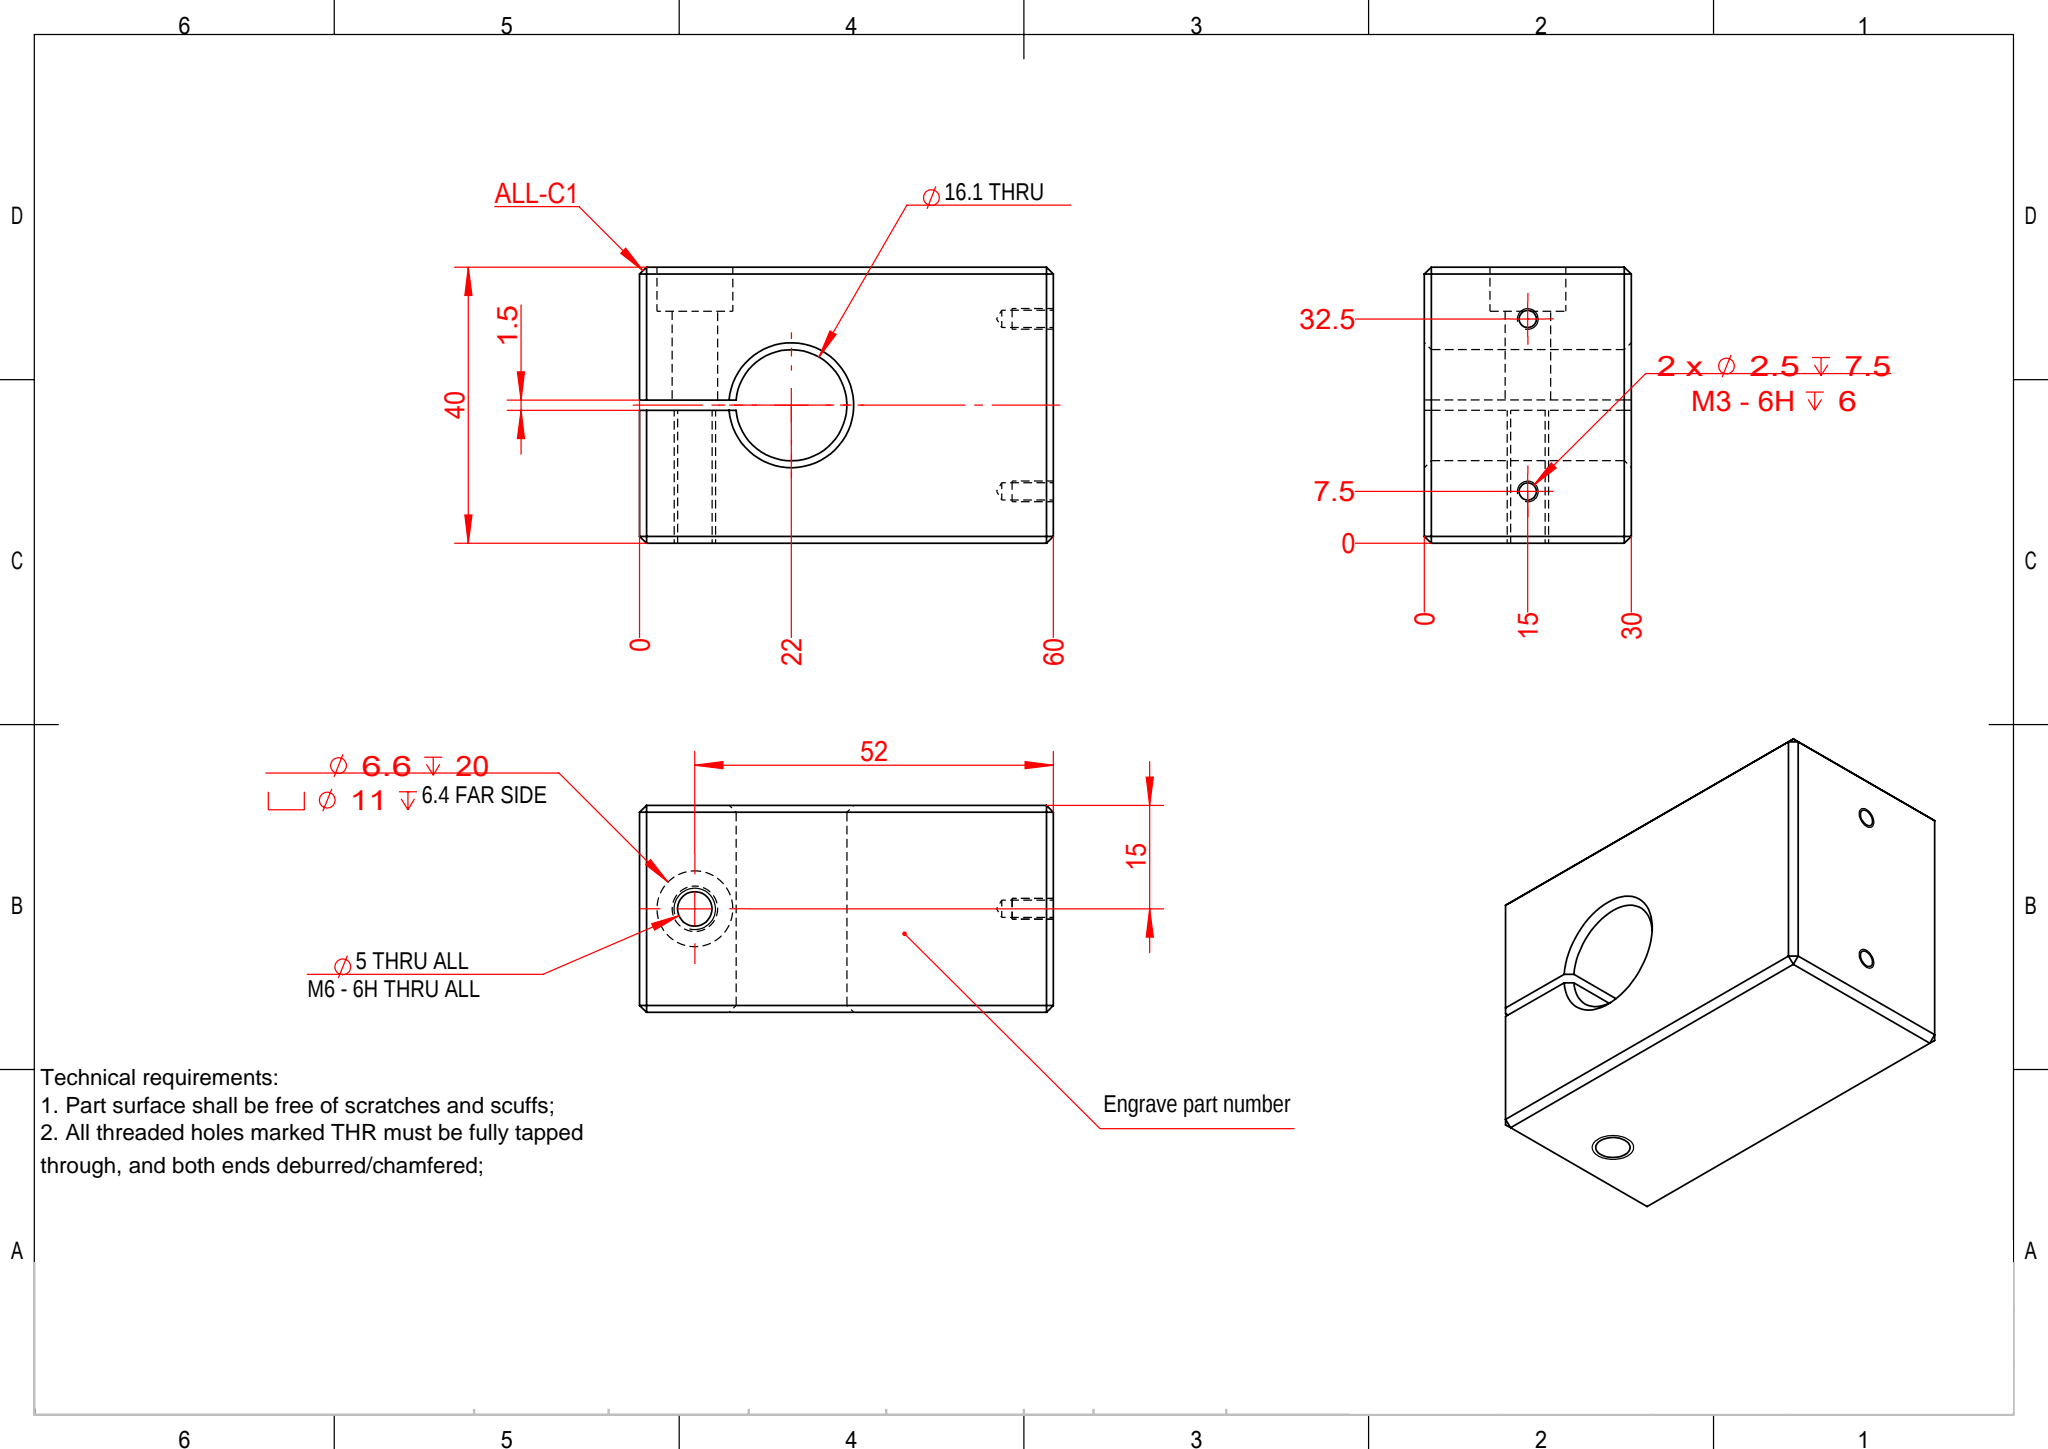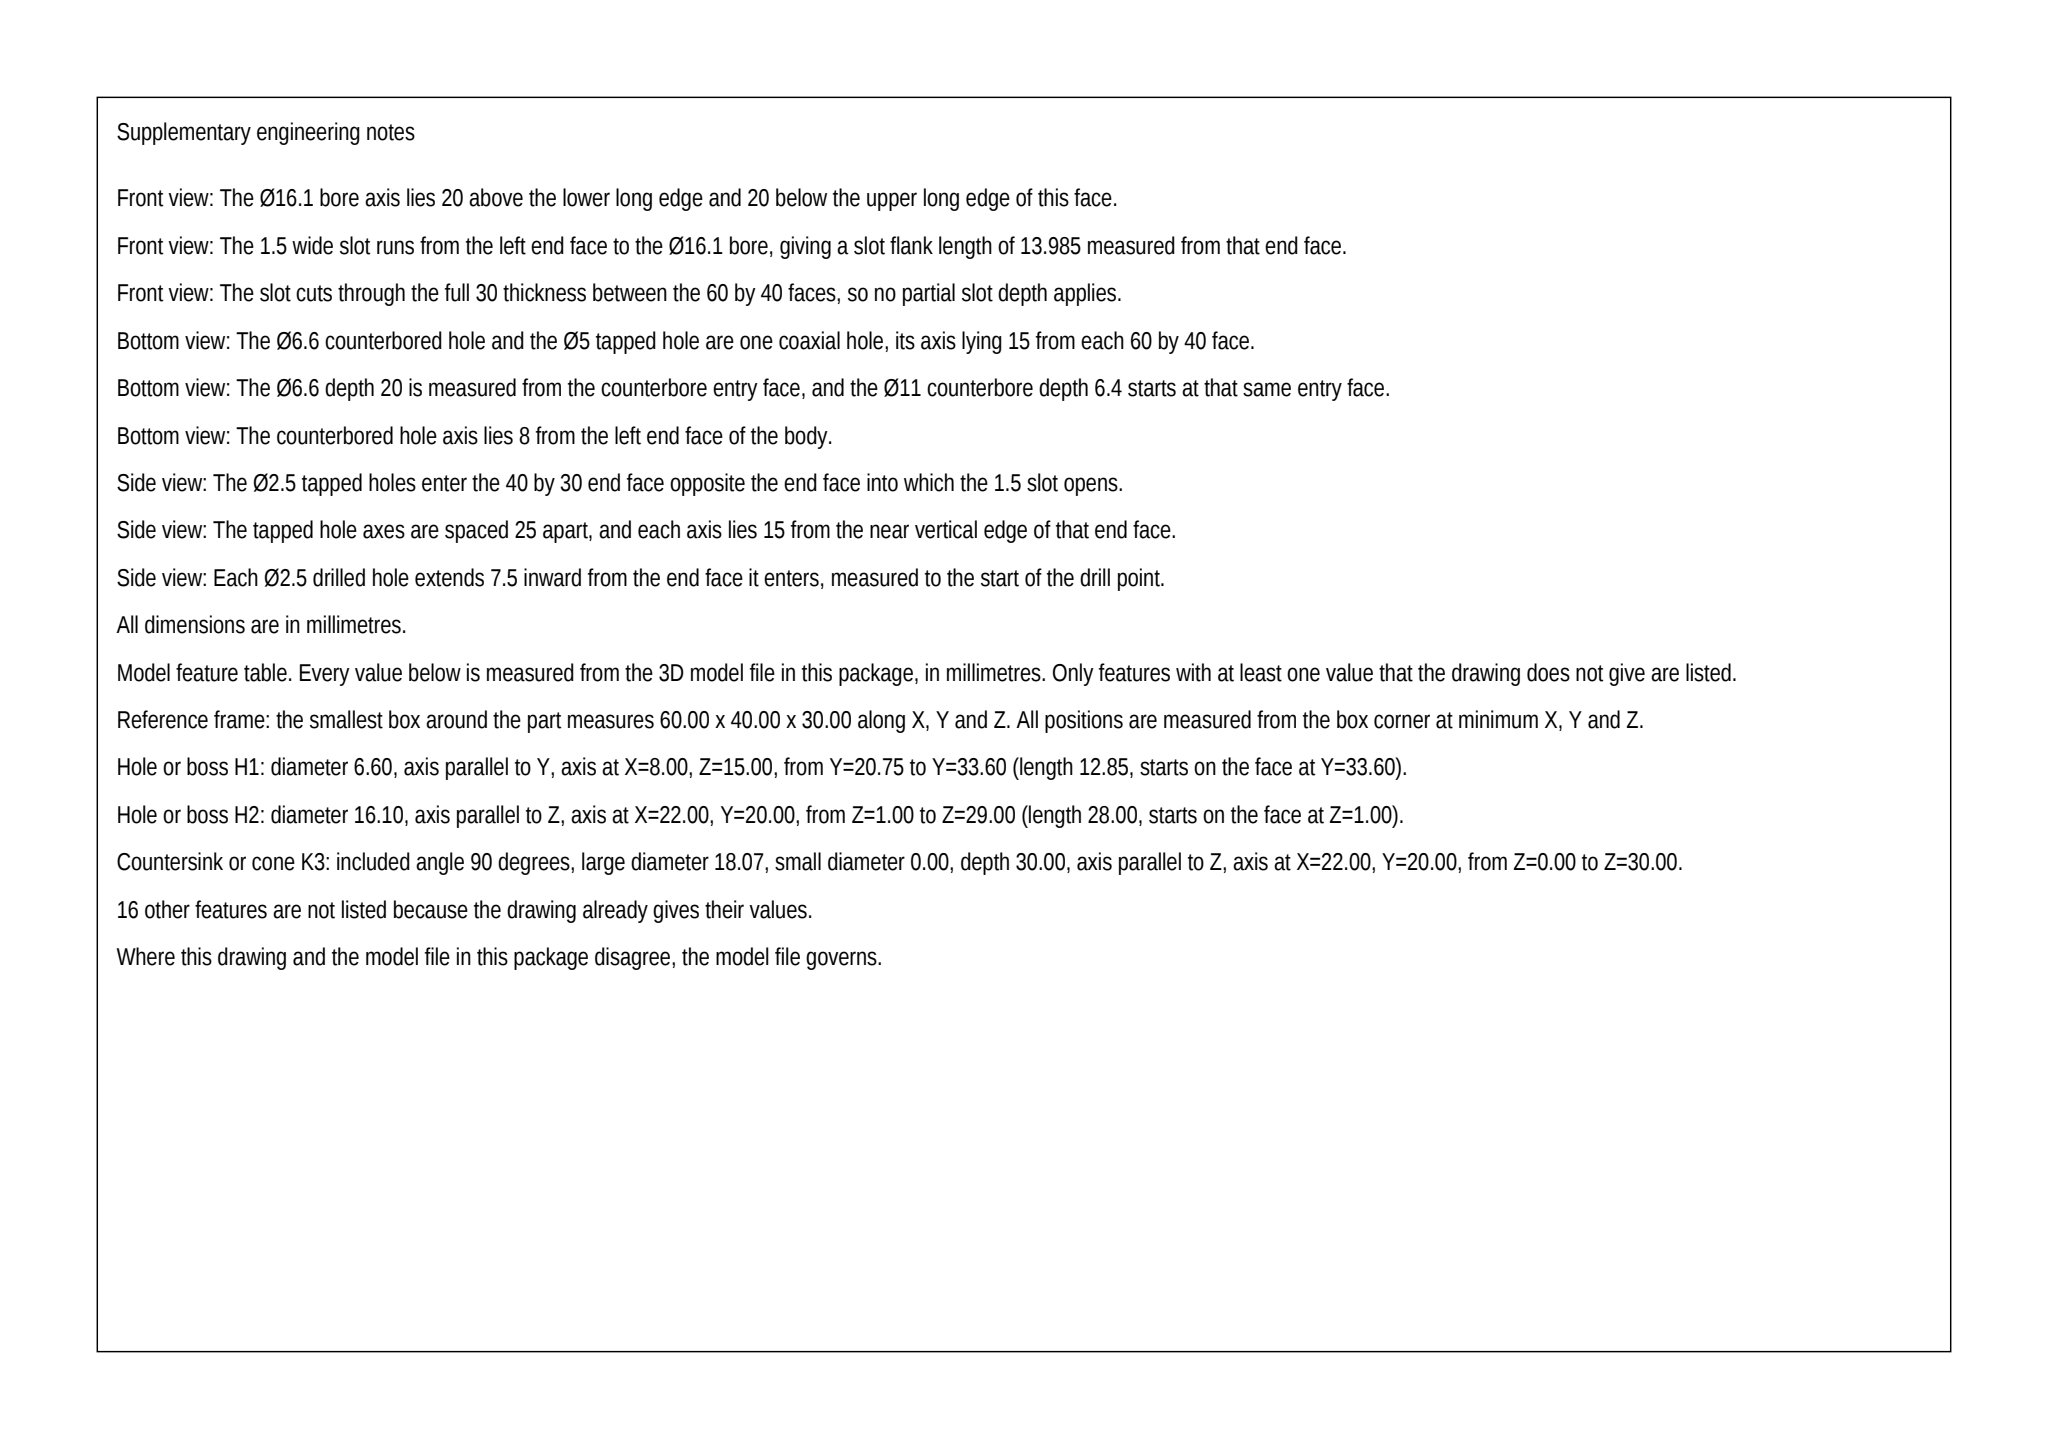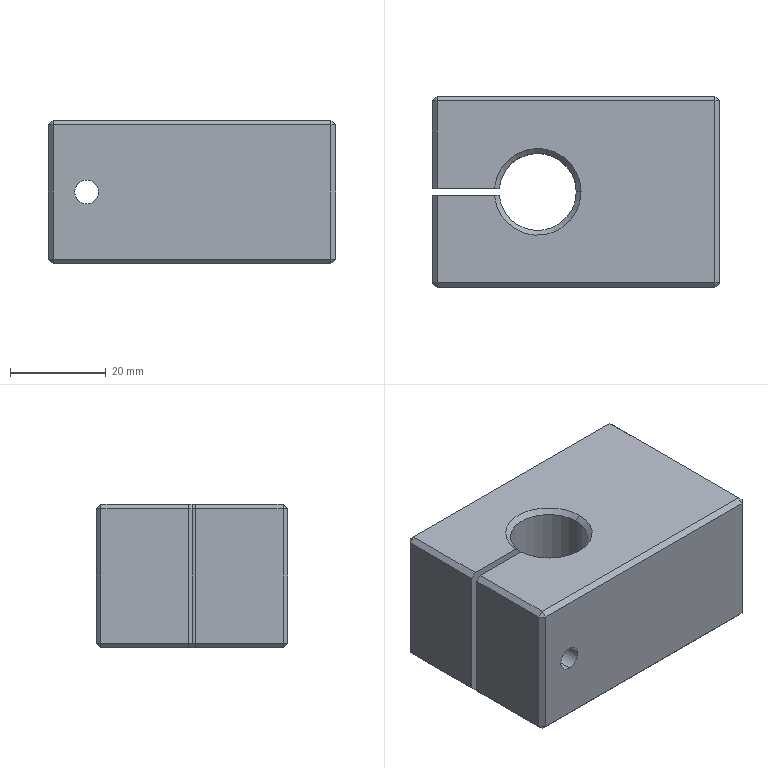Part | SolidWorks | mm | 1 solid | 51 faces | box 60 x 40 x 30 mm | volume 63458 mm3 | plane 32 | cylinder 12 | cone 7 | commonest cylinder face diameters 2.5 x4 5 x2 11 x2 6.6 x2 16.1 x2
build123d program:
from build123d import *

# Parameters (mm, degrees)
SKETCH1_W                                       = 60
SKETCH1_H                                       = 40
BOSS_EXTRUDE1_DEPTH                             = 30
SKETCH2_R                                       = 8.05
CUT_EXTRUDE1_DEPTH                              = 79.102
CHAMFER1_SIZE                                   = 1
SKETCH3_W                                       = 34.45
SKETCH3_H                                       = 1.5
CUT_EXTRUDE2_DEPTH                              = 79.102
M6_HEX_SOCKET_HEAD_CAP_SCREW_CBORE1_D           = 6.6
M6_HEX_SOCKET_HEAD_CAP_SCREW_CBORE1_DEPTH       = 20
M6_HEX_SOCKET_HEAD_CAP_SCREW_CBORE1_CBORE_D     = 11
M6_HEX_SOCKET_HEAD_CAP_SCREW_CBORE1_CBORE_DEPTH = 6.4
M6_HEX_SOCKET_HEAD_CAP_SCREW_CBORE1_TIP         = 1.983
M6_TAPPED_HOLE1_D                               = 5
M3_TAPPED_HOLE1_D                               = 2.5
M3_TAPPED_HOLE1_DEPTH                           = 7.5
M3_TAPPED_HOLE1_TIP                             = 0.7511


with BuildPart() as part:
    # Sketch1 → Boss-Extrude1 (new body)
    with BuildSketch(Plane.XY):
        with Locations((30, 20)):
            Rectangle(SKETCH1_W, SKETCH1_H)
    extrude(amount=BOSS_EXTRUDE1_DEPTH)

    # Sketch2 → Cut-Extrude1 (cut, through all)
    with BuildSketch(Plane.XY.offset(30)):
        with Locations((22, 20)):
            Circle(SKETCH2_R)
    extrude(amount=-CUT_EXTRUDE1_DEPTH, mode=Mode.SUBTRACT)

    # Chamfer1
    chamfer1_edges = [part.edges().sort_by_distance(p)[0] for p in [
        (60, 20, 30),
        (30, 40, 30),
        (13.95, 20, 0),
        (13.95, 20, 30),
        (0, 20, 30),
        (30, 40, 0),
        (60, 20, 0),
        (30, 0, 0),
        (0, 20, 0),
        (30, 0, 30),
        (0, 40, 15),
        (60, 40, 15),
        (60, 0, 15),
        (0, 0, 15),
    ]]
    chamfer(chamfer1_edges, length=CHAMFER1_SIZE)

    # Sketch3 → Cut-Extrude2 (cut, through all)
    with BuildSketch(Plane.XY.offset(30)):
        with Locations((2.279, 20)):
            Rectangle(SKETCH3_W, SKETCH3_H)
    extrude(amount=-CUT_EXTRUDE2_DEPTH, mode=Mode.SUBTRACT)

    # M6 Hex Socket Head Cap Screw CBORE1
    with Locations(Plane(origin=(0, 40, 0), x_dir=(1, 0, 0), z_dir=(0, 1, 0))):
        with Locations((8, -15)):
            CounterBoreHole(M6_HEX_SOCKET_HEAD_CAP_SCREW_CBORE1_D / 2, M6_HEX_SOCKET_HEAD_CAP_SCREW_CBORE1_CBORE_D / 2, M6_HEX_SOCKET_HEAD_CAP_SCREW_CBORE1_CBORE_DEPTH, depth=M6_HEX_SOCKET_HEAD_CAP_SCREW_CBORE1_DEPTH)
            with Locations((0, 0, -(M6_HEX_SOCKET_HEAD_CAP_SCREW_CBORE1_DEPTH + M6_HEX_SOCKET_HEAD_CAP_SCREW_CBORE1_TIP / 2))):  # 118° drill point
                Cone(0, M6_HEX_SOCKET_HEAD_CAP_SCREW_CBORE1_D / 2, M6_HEX_SOCKET_HEAD_CAP_SCREW_CBORE1_TIP, mode=Mode.SUBTRACT)

    # M6 Tapped Hole1 (through all)
    with Locations(Plane(origin=(0, 0, 0), x_dir=(-1, 0, 0), z_dir=(0, -1, 0))):
        with Locations((-8, -15)):
            Hole(M6_TAPPED_HOLE1_D / 2)

    # M3 Tapped Hole1
    with Locations(Plane(origin=(60, 0, 0), x_dir=(0, 0, -1), z_dir=(1, 0, 0))):
        with Locations((-15, 32.5), (-15, 7.5)):
            Hole(M3_TAPPED_HOLE1_D / 2, depth=M3_TAPPED_HOLE1_DEPTH)
            with Locations((0, 0, -(M3_TAPPED_HOLE1_DEPTH + M3_TAPPED_HOLE1_TIP / 2))):  # 118° drill point
                Cone(0, M3_TAPPED_HOLE1_D / 2, M3_TAPPED_HOLE1_TIP, mode=Mode.SUBTRACT)


solid = part.part